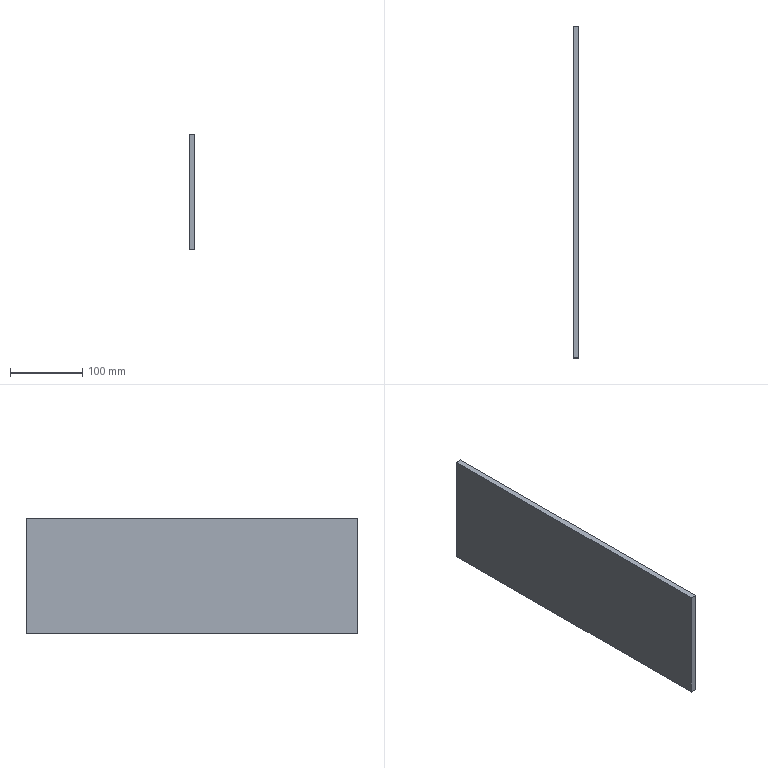Component | SolidWorks | VerticalPlate-1 | 1 solid | 6 faces | box 8 x 460 x 160 mm | volume 588800 mm3 | plane 6
build123d program:
from build123d import *

# Parameters (mm, degrees)
SKETCH1_W           = 160
SKETCH1_H           = 460
BOSS_EXTRUDE1_DEPTH = 4


with BuildPart() as part:
    # Sketch1 → Boss-Extrude1 (new, symmetric)
    with BuildSketch(Plane.XY):
        Rectangle(SKETCH1_W, SKETCH1_H)
    extrude(amount=BOSS_EXTRUDE1_DEPTH, both=True)


solid = part.part

# Placed as in the assembly
solid = solid.moved(Location((41.398, 237.837, 100), (0, 90, 0)))
STEP:
#1=COLOUR_RGB('',0.7922,0.8196,0.9333);
#2=FILL_AREA_STYLE_COLOUR('',#1);
#3=FILL_AREA_STYLE('',(#2));
#4=SURFACE_STYLE_FILL_AREA(#3);
#5=SURFACE_SIDE_STYLE('',(#4));
#6=SURFACE_STYLE_USAGE(.BOTH.,#5);
#7=PRESENTATION_STYLE_ASSIGNMENT((#6));
#8=CARTESIAN_POINT('',(1.787,18.419,0.7874));
#9=VERTEX_POINT('',#8);
#10=CARTESIAN_POINT('',(1.787,0.3085,0.7874));
#11=VERTEX_POINT('',#10);
#12=CARTESIAN_POINT('',(1.787,0.3085,0.7874));
#13=DIRECTION('',(0.,-1.,0.));
#14=VECTOR('',#13,39.37);
#15=LINE('',#12,#14);
#16=EDGE_CURVE('',#9,#11,#15,.T.);
#17=ORIENTED_EDGE('',*,*,#16,.T.);
#18=CARTESIAN_POINT('',(1.472,0.3085,0.7874));
#19=VERTEX_POINT('',#18);
#20=CARTESIAN_POINT('',(1.472,0.3085,0.7874));
#21=DIRECTION('',(1.,0.,0.));
#22=VECTOR('',#21,39.37);
#23=LINE('',#20,#22);
#24=EDGE_CURVE('',#19,#11,#23,.T.);
#25=ORIENTED_EDGE('',*,*,#24,.F.);
#26=CARTESIAN_POINT('',(1.472,18.419,0.7874));
#27=VERTEX_POINT('',#26);
#28=CARTESIAN_POINT('',(1.472,0.3085,0.7874));
#29=DIRECTION('',(0.,-1.,0.));
#30=VECTOR('',#29,39.37);
#31=LINE('',#28,#30);
#32=EDGE_CURVE('',#27,#19,#31,.T.);
#33=ORIENTED_EDGE('',*,*,#32,.F.);
#34=CARTESIAN_POINT('',(1.472,18.419,0.7874));
#35=DIRECTION('',(1.,0.,0.));
#36=VECTOR('',#35,39.37);
#37=LINE('',#34,#36);
#38=EDGE_CURVE('',#27,#9,#37,.T.);
#39=ORIENTED_EDGE('',*,*,#38,.T.);
#40=EDGE_LOOP('',(#17,#25,#33,#39));
#41=FACE_OUTER_BOUND('',#40,.T.);
#42=CARTESIAN_POINT('',(1.472,0.3085,0.7874));
#43=DIRECTION('',(0.,0.,1.));
#44=DIRECTION('',(1.,0.,0.));
#45=AXIS2_PLACEMENT_3D('',#42,#43,#44);
#46=PLANE('',#45);
#47=ADVANCED_FACE('',(#41),#46,.F.);
#48=CARTESIAN_POINT('',(1.787,0.3085,7.087));
#49=VERTEX_POINT('',#48);
#50=CARTESIAN_POINT('',(1.787,0.3085,7.087));
#51=DIRECTION('',(0.,0.,1.));
#52=VECTOR('',#51,39.37);
#53=LINE('',#50,#52);
#54=EDGE_CURVE('',#11,#49,#53,.T.);
#55=ORIENTED_EDGE('',*,*,#54,.T.);
#56=CARTESIAN_POINT('',(1.472,0.3085,7.087));
#57=VERTEX_POINT('',#56);
#58=CARTESIAN_POINT('',(1.472,0.3085,7.087));
#59=DIRECTION('',(1.,0.,0.));
#60=VECTOR('',#59,39.37);
#61=LINE('',#58,#60);
#62=EDGE_CURVE('',#57,#49,#61,.T.);
#63=ORIENTED_EDGE('',*,*,#62,.F.);
#64=CARTESIAN_POINT('',(1.472,0.3085,7.087));
#65=DIRECTION('',(0.,0.,1.));
#66=VECTOR('',#65,39.37);
#67=LINE('',#64,#66);
#68=EDGE_CURVE('',#19,#57,#67,.T.);
#69=ORIENTED_EDGE('',*,*,#68,.F.);
#70=ORIENTED_EDGE('',*,*,#24,.T.);
#71=EDGE_LOOP('',(#55,#63,#69,#70));
#72=FACE_OUTER_BOUND('',#71,.T.);
#73=CARTESIAN_POINT('',(1.472,0.3085,7.087));
#74=DIRECTION('',(0.,1.,0.));
#75=DIRECTION('',(-1.,0.,0.));
#76=AXIS2_PLACEMENT_3D('',#73,#74,#75);
#77=PLANE('',#76);
#78=ADVANCED_FACE('',(#72),#77,.F.);
#79=CARTESIAN_POINT('',(1.787,18.419,7.087));
#80=VERTEX_POINT('',#79);
#81=CARTESIAN_POINT('',(1.787,0.3085,7.087));
#82=DIRECTION('',(0.,1.,0.));
#83=VECTOR('',#82,39.37);
#84=LINE('',#81,#83);
#85=EDGE_CURVE('',#49,#80,#84,.T.);
#86=ORIENTED_EDGE('',*,*,#85,.T.);
#87=CARTESIAN_POINT('',(1.472,18.419,7.087));
#88=VERTEX_POINT('',#87);
#89=CARTESIAN_POINT('',(1.472,18.419,7.087));
#90=DIRECTION('',(1.,0.,0.));
#91=VECTOR('',#90,39.37);
#92=LINE('',#89,#91);
#93=EDGE_CURVE('',#88,#80,#92,.T.);
#94=ORIENTED_EDGE('',*,*,#93,.F.);
#95=CARTESIAN_POINT('',(1.472,0.3085,7.087));
#96=DIRECTION('',(0.,1.,0.));
#97=VECTOR('',#96,39.37);
#98=LINE('',#95,#97);
#99=EDGE_CURVE('',#57,#88,#98,.T.);
#100=ORIENTED_EDGE('',*,*,#99,.F.);
#101=ORIENTED_EDGE('',*,*,#62,.T.);
#102=EDGE_LOOP('',(#86,#94,#100,#101));
#103=FACE_OUTER_BOUND('',#102,.T.);
#104=CARTESIAN_POINT('',(1.472,0.3085,7.087));
#105=DIRECTION('',(0.,0.,-1.));
#106=DIRECTION('',(-1.,0.,0.));
#107=AXIS2_PLACEMENT_3D('',#104,#105,#106);
#108=PLANE('',#107);
#109=ADVANCED_FACE('',(#103),#108,.F.);
#110=CARTESIAN_POINT('',(1.787,18.419,7.087));
#111=DIRECTION('',(0.,0.,-1.));
#112=VECTOR('',#111,39.37);
#113=LINE('',#110,#112);
#114=EDGE_CURVE('',#80,#9,#113,.T.);
#115=ORIENTED_EDGE('',*,*,#114,.T.);
#116=ORIENTED_EDGE('',*,*,#38,.F.);
#117=CARTESIAN_POINT('',(1.472,18.419,7.087));
#118=DIRECTION('',(0.,0.,-1.));
#119=VECTOR('',#118,39.37);
#120=LINE('',#117,#119);
#121=EDGE_CURVE('',#88,#27,#120,.T.);
#122=ORIENTED_EDGE('',*,*,#121,.F.);
#123=ORIENTED_EDGE('',*,*,#93,.T.);
#124=EDGE_LOOP('',(#115,#116,#122,#123));
#125=FACE_OUTER_BOUND('',#124,.T.);
#126=CARTESIAN_POINT('',(1.472,18.419,7.087));
#127=DIRECTION('',(0.,-1.,0.));
#128=DIRECTION('',(1.,0.,0.));
#129=AXIS2_PLACEMENT_3D('',#126,#127,#128);
#130=PLANE('',#129);
#131=ADVANCED_FACE('',(#125),#130,.F.);
#132=ORIENTED_EDGE('',*,*,#32,.T.);
#133=ORIENTED_EDGE('',*,*,#68,.T.);
#134=ORIENTED_EDGE('',*,*,#99,.T.);
#135=ORIENTED_EDGE('',*,*,#121,.T.);
#136=EDGE_LOOP('',(#132,#133,#134,#135));
#137=FACE_OUTER_BOUND('',#136,.T.);
#138=CARTESIAN_POINT('',(1.472,9.364,3.937));
#139=DIRECTION('',(-1.,0.,0.));
#140=DIRECTION('',(0.,0.,1.));
#141=AXIS2_PLACEMENT_3D('',#138,#139,#140);
#142=PLANE('',#141);
#143=ADVANCED_FACE('',(#137),#142,.T.);
#144=ORIENTED_EDGE('',*,*,#16,.F.);
#145=ORIENTED_EDGE('',*,*,#114,.F.);
#146=ORIENTED_EDGE('',*,*,#85,.F.);
#147=ORIENTED_EDGE('',*,*,#54,.F.);
#148=EDGE_LOOP('',(#144,#145,#146,#147));
#149=FACE_OUTER_BOUND('',#148,.T.);
#150=CARTESIAN_POINT('',(1.787,9.364,3.937));
#151=DIRECTION('',(-1.,0.,0.));
#152=DIRECTION('',(0.,0.,1.));
#153=AXIS2_PLACEMENT_3D('',#150,#151,#152);
#154=PLANE('',#153);
#155=ADVANCED_FACE('',(#149),#154,.F.);
#156=CLOSED_SHELL('',(#47,#78,#109,#131,#143,#155));
#157=MANIFOLD_SOLID_BREP('',#156);
#158=STYLED_ITEM('',(#7),#157);
#159=PRESENTATION_LAYER_ASSIGNMENT('','',(#158));
#160=CARTESIAN_POINT('',(0.,0.,0.));
#161=DIRECTION('',(0.,0.,1.));
#162=DIRECTION('',(1.,0.,0.));
#163=AXIS2_PLACEMENT_3D('',#160,#161,#162);
#164=(LENGTH_UNIT()NAMED_UNIT(*)SI_UNIT($,.METRE.));
#165=LENGTH_MEASURE_WITH_UNIT(LENGTH_MEASURE(0.0254),#164);
#166=DIMENSIONAL_EXPONENTS(1.,0.,0.,0.,0.,0.,0.);
#167=(CONVERSION_BASED_UNIT('',#165)LENGTH_UNIT()NAMED_UNIT(#166));
#168=UNCERTAINTY_MEASURE_WITH_UNIT(LENGTH_MEASURE(0.00001),#167,'','');
#169=(NAMED_UNIT(*)PLANE_ANGLE_UNIT()SI_UNIT($,.RADIAN.));
#170=(NAMED_UNIT(*)SI_UNIT($,.STERADIAN.)SOLID_ANGLE_UNIT());
#171=(GEOMETRIC_REPRESENTATION_CONTEXT(3)GLOBAL_UNCERTAINTY_ASSIGNED_CONTEXT((#168))GLOBAL_UNIT_ASSIGNED_CONTEXT((#167,#169,#170))REPRESENTATION_CONTEXT('',''));
#172=ADVANCED_BREP_SHAPE_REPRESENTATION('',(#157,#163),#171);
#173=(LENGTH_UNIT()NAMED_UNIT(*)SI_UNIT($,.METRE.));
#174=LENGTH_MEASURE_WITH_UNIT(LENGTH_MEASURE(0.0254),#173);
#175=DIMENSIONAL_EXPONENTS(1.,0.,0.,0.,0.,0.,0.);
#176=(CONVERSION_BASED_UNIT('',#174)LENGTH_UNIT()NAMED_UNIT(#175));
#177=UNCERTAINTY_MEASURE_WITH_UNIT(LENGTH_MEASURE(0.00001),#176,'','');
#178=(NAMED_UNIT(*)PLANE_ANGLE_UNIT()SI_UNIT($,.RADIAN.));
#179=(NAMED_UNIT(*)SI_UNIT($,.STERADIAN.)SOLID_ANGLE_UNIT());
#180=(GEOMETRIC_REPRESENTATION_CONTEXT(3)GLOBAL_UNCERTAINTY_ASSIGNED_CONTEXT((#177))GLOBAL_UNIT_ASSIGNED_CONTEXT((#176,#178,#179))REPRESENTATION_CONTEXT('',''));
#181=MECHANICAL_DESIGN_GEOMETRIC_PRESENTATION_REPRESENTATION('',(#158),#180);